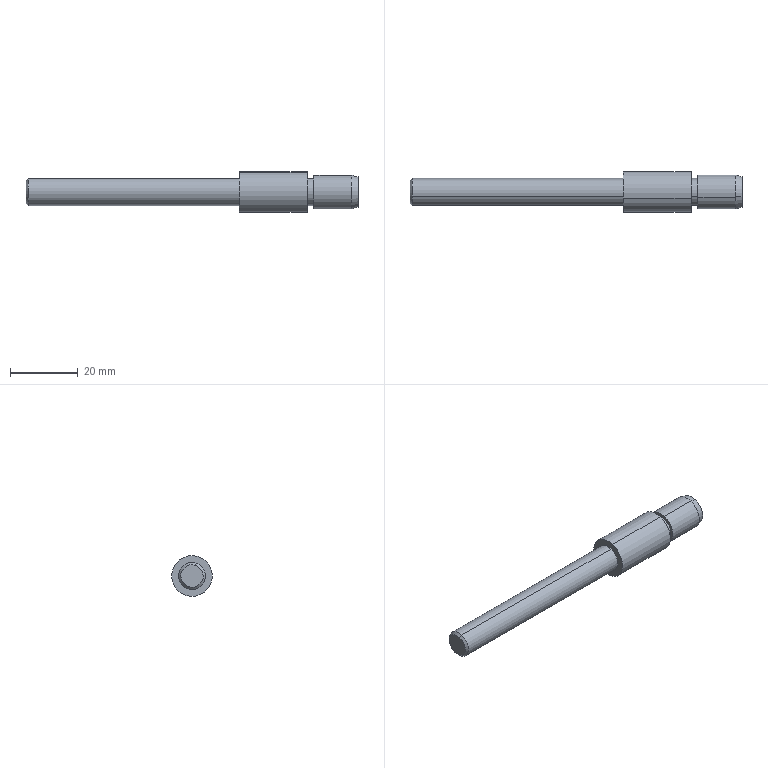Component | SolidWorks | 10Pin-1 | 1 solid | 17 faces | box 98 x 12 x 12 mm | volume 6529 mm3 | cylinder 8 | plane 5 | cone 4 | commonest cylinder face diameters 8 x4 10 x2 12 x2
STEP:
#1=COLOUR_RGB('',0.7922,0.8196,0.9333);
#2=FILL_AREA_STYLE_COLOUR('',#1);
#3=FILL_AREA_STYLE('',(#2));
#4=SURFACE_STYLE_FILL_AREA(#3);
#5=SURFACE_SIDE_STYLE('',(#4));
#6=SURFACE_STYLE_USAGE(.BOTH.,#5);
#7=PRESENTATION_STYLE_ASSIGNMENT((#6));
#8=CARTESIAN_POINT('',(-15.354,4.369,-0.1755));
#9=VERTEX_POINT('',#8);
#10=CARTESIAN_POINT('',(-15.354,4.291,0.07414));
#11=VERTEX_POINT('',#10);
#12=CARTESIAN_POINT('',(-15.354,4.33,-0.05068));
#13=DIRECTION('',(1.,0.,0.));
#14=DIRECTION('',(0.,0.3,-0.9539));
#15=AXIS2_PLACEMENT_3D('',#12,#13,#14);
#16=CIRCLE('',#15,0.1308);
#17=EDGE_CURVE('',#9,#11,#16,.T.);
#18=ORIENTED_EDGE('',*,*,#17,.T.);
#19=CARTESIAN_POINT('',(-15.328,4.283,0.09955));
#20=VERTEX_POINT('',#19);
#21=CARTESIAN_POINT('',(-15.354,4.291,0.07414));
#22=DIRECTION('',(0.7071,-0.2121,0.6745));
#23=VECTOR('',#22,39.37);
#24=LINE('',#21,#23);
#25=EDGE_CURVE('',#11,#20,#24,.T.);
#26=ORIENTED_EDGE('',*,*,#25,.T.);
#27=CARTESIAN_POINT('',(-15.328,4.377,-0.2009));
#28=VERTEX_POINT('',#27);
#29=CARTESIAN_POINT('',(-15.328,4.33,-0.05068));
#30=DIRECTION('',(1.,0.,0.));
#31=DIRECTION('',(0.,0.3,-0.9539));
#32=AXIS2_PLACEMENT_3D('',#29,#30,#31);
#33=CIRCLE('',#32,0.1575);
#34=EDGE_CURVE('',#28,#20,#33,.T.);
#35=ORIENTED_EDGE('',*,*,#34,.F.);
#36=CARTESIAN_POINT('',(-15.354,4.369,-0.1755));
#37=DIRECTION('',(0.7071,0.2121,-0.6745));
#38=VECTOR('',#37,39.37);
#39=LINE('',#36,#38);
#40=EDGE_CURVE('',#9,#28,#39,.T.);
#41=ORIENTED_EDGE('',*,*,#40,.F.);
#42=EDGE_LOOP('',(#18,#26,#35,#41));
#43=FACE_OUTER_BOUND('',#42,.T.);
#44=CARTESIAN_POINT('',(-15.354,4.33,-0.05068));
#45=DIRECTION('',(1.,0.,0.));
#46=DIRECTION('',(0.,0.3,-0.9539));
#47=AXIS2_PLACEMENT_3D('',#44,#45,#46);
#48=CONICAL_SURFACE('',#47,0.1308,0.7854);
#49=ADVANCED_FACE('',(#43),#48,.T.);
#50=CARTESIAN_POINT('',(-11.496,4.383,-0.2183));
#51=VERTEX_POINT('',#50);
#52=CARTESIAN_POINT('',(-11.496,4.277,0.117));
#53=VERTEX_POINT('',#52);
#54=CARTESIAN_POINT('',(-11.496,4.33,-0.05068));
#55=DIRECTION('',(1.,0.,0.));
#56=DIRECTION('',(0.,0.3,-0.9539));
#57=AXIS2_PLACEMENT_3D('',#54,#55,#56);
#58=CIRCLE('',#57,0.1758);
#59=EDGE_CURVE('',#51,#53,#58,.T.);
#60=ORIENTED_EDGE('',*,*,#59,.F.);
#61=CARTESIAN_POINT('',(-11.575,4.389,-0.2385));
#62=VERTEX_POINT('',#61);
#63=CARTESIAN_POINT('',(-11.496,4.383,-0.2183));
#64=DIRECTION('',(-0.9659,0.07764,-0.2469));
#65=VECTOR('',#64,39.37);
#66=LINE('',#63,#65);
#67=EDGE_CURVE('',#51,#62,#66,.T.);
#68=ORIENTED_EDGE('',*,*,#67,.T.);
#69=CARTESIAN_POINT('',(-11.575,4.271,0.1371));
#70=VERTEX_POINT('',#69);
#71=CARTESIAN_POINT('',(-11.575,4.33,-0.05068));
#72=DIRECTION('',(-1.,-0.,-0.));
#73=DIRECTION('',(0.,0.3,-0.9539));
#74=AXIS2_PLACEMENT_3D('',#71,#72,#73);
#75=CIRCLE('',#74,0.1969);
#76=EDGE_CURVE('',#70,#62,#75,.T.);
#77=ORIENTED_EDGE('',*,*,#76,.F.);
#78=CARTESIAN_POINT('',(-11.496,4.277,0.117));
#79=DIRECTION('',(-0.9659,-0.07764,0.2469));
#80=VECTOR('',#79,39.37);
#81=LINE('',#78,#80);
#82=EDGE_CURVE('',#53,#70,#81,.T.);
#83=ORIENTED_EDGE('',*,*,#82,.F.);
#84=EDGE_LOOP('',(#60,#68,#77,#83));
#85=FACE_OUTER_BOUND('',#84,.T.);
#86=CARTESIAN_POINT('',(-11.496,4.33,-0.05068));
#87=DIRECTION('',(-1.,-0.,-0.));
#88=DIRECTION('',(0.,-0.3,0.9539));
#89=AXIS2_PLACEMENT_3D('',#86,#87,#88);
#90=CONICAL_SURFACE('',#89,0.1758,0.2618);
#91=ADVANCED_FACE('',(#85),#90,.T.);
#92=ORIENTED_EDGE('',*,*,#76,.T.);
#93=CARTESIAN_POINT('',(-12.008,4.389,-0.2385));
#94=VERTEX_POINT('',#93);
#95=CARTESIAN_POINT('',(-11.496,4.389,-0.2385));
#96=DIRECTION('',(-1.,-0.,-0.));
#97=VECTOR('',#96,39.37);
#98=LINE('',#95,#97);
#99=EDGE_CURVE('',#62,#94,#98,.T.);
#100=ORIENTED_EDGE('',*,*,#99,.T.);
#101=CARTESIAN_POINT('',(-12.008,4.271,0.1371));
#102=VERTEX_POINT('',#101);
#103=CARTESIAN_POINT('',(-12.008,4.33,-0.05068));
#104=DIRECTION('',(1.,0.,0.));
#105=DIRECTION('',(0.,0.3,-0.9539));
#106=AXIS2_PLACEMENT_3D('',#103,#104,#105);
#107=CIRCLE('',#106,0.1969);
#108=EDGE_CURVE('',#94,#102,#107,.T.);
#109=ORIENTED_EDGE('',*,*,#108,.T.);
#110=CARTESIAN_POINT('',(-11.496,4.271,0.1371));
#111=DIRECTION('',(-1.,-0.,-0.));
#112=VECTOR('',#111,39.37);
#113=LINE('',#110,#112);
#114=EDGE_CURVE('',#70,#102,#113,.T.);
#115=ORIENTED_EDGE('',*,*,#114,.F.);
#116=EDGE_LOOP('',(#92,#100,#109,#115));
#117=FACE_OUTER_BOUND('',#116,.T.);
#118=CARTESIAN_POINT('',(-11.496,4.33,-0.05068));
#119=DIRECTION('',(-1.,-0.,-0.));
#120=DIRECTION('',(0.,-0.3,0.9539));
#121=AXIS2_PLACEMENT_3D('',#118,#119,#120);
#122=CYLINDRICAL_SURFACE('',#121,0.1969);
#123=ADVANCED_FACE('',(#117),#122,.T.);
#124=CARTESIAN_POINT('',(-12.008,4.377,-0.2009));
#125=VERTEX_POINT('',#124);
#126=CARTESIAN_POINT('',(-12.008,4.283,0.09955));
#127=VERTEX_POINT('',#126);
#128=CARTESIAN_POINT('',(-12.008,4.33,-0.05068));
#129=DIRECTION('',(1.,0.,0.));
#130=DIRECTION('',(0.,0.3,-0.9539));
#131=AXIS2_PLACEMENT_3D('',#128,#129,#130);
#132=CIRCLE('',#131,0.1575);
#133=EDGE_CURVE('',#125,#127,#132,.T.);
#134=ORIENTED_EDGE('',*,*,#133,.F.);
#135=CARTESIAN_POINT('',(-12.087,4.377,-0.2009));
#136=VERTEX_POINT('',#135);
#137=CARTESIAN_POINT('',(-12.008,4.377,-0.2009));
#138=DIRECTION('',(-1.,-0.,-0.));
#139=VECTOR('',#138,39.37);
#140=LINE('',#137,#139);
#141=EDGE_CURVE('',#125,#136,#140,.T.);
#142=ORIENTED_EDGE('',*,*,#141,.T.);
#143=CARTESIAN_POINT('',(-12.087,4.283,0.09955));
#144=VERTEX_POINT('',#143);
#145=CARTESIAN_POINT('',(-12.087,4.33,-0.05068));
#146=DIRECTION('',(1.,0.,0.));
#147=DIRECTION('',(0.,0.3,-0.9539));
#148=AXIS2_PLACEMENT_3D('',#145,#146,#147);
#149=CIRCLE('',#148,0.1575);
#150=EDGE_CURVE('',#136,#144,#149,.T.);
#151=ORIENTED_EDGE('',*,*,#150,.T.);
#152=CARTESIAN_POINT('',(-12.008,4.283,0.09955));
#153=DIRECTION('',(-1.,-0.,-0.));
#154=VECTOR('',#153,39.37);
#155=LINE('',#152,#154);
#156=EDGE_CURVE('',#127,#144,#155,.T.);
#157=ORIENTED_EDGE('',*,*,#156,.F.);
#158=EDGE_LOOP('',(#134,#142,#151,#157));
#159=FACE_OUTER_BOUND('',#158,.T.);
#160=CARTESIAN_POINT('',(-12.008,4.33,-0.05068));
#161=DIRECTION('',(-1.,-0.,-0.));
#162=DIRECTION('',(0.,-0.3,0.9539));
#163=AXIS2_PLACEMENT_3D('',#160,#161,#162);
#164=CYLINDRICAL_SURFACE('',#163,0.1575);
#165=ADVANCED_FACE('',(#159),#164,.T.);
#166=CARTESIAN_POINT('',(-12.087,4.401,-0.276));
#167=VERTEX_POINT('',#166);
#168=CARTESIAN_POINT('',(-12.087,4.259,0.1747));
#169=VERTEX_POINT('',#168);
#170=CARTESIAN_POINT('',(-12.087,4.33,-0.05068));
#171=DIRECTION('',(1.,0.,0.));
#172=DIRECTION('',(0.,0.3,-0.9539));
#173=AXIS2_PLACEMENT_3D('',#170,#171,#172);
#174=CIRCLE('',#173,0.2362);
#175=EDGE_CURVE('',#167,#169,#174,.T.);
#176=ORIENTED_EDGE('',*,*,#175,.F.);
#177=CARTESIAN_POINT('',(-12.874,4.401,-0.276));
#178=VERTEX_POINT('',#177);
#179=CARTESIAN_POINT('',(-12.087,4.401,-0.276));
#180=DIRECTION('',(-1.,-0.,-0.));
#181=VECTOR('',#180,39.37);
#182=LINE('',#179,#181);
#183=EDGE_CURVE('',#167,#178,#182,.T.);
#184=ORIENTED_EDGE('',*,*,#183,.T.);
#185=CARTESIAN_POINT('',(-12.874,4.259,0.1747));
#186=VERTEX_POINT('',#185);
#187=CARTESIAN_POINT('',(-12.874,4.33,-0.05068));
#188=DIRECTION('',(1.,0.,0.));
#189=DIRECTION('',(0.,0.3,-0.9539));
#190=AXIS2_PLACEMENT_3D('',#187,#188,#189);
#191=CIRCLE('',#190,0.2362);
#192=EDGE_CURVE('',#178,#186,#191,.T.);
#193=ORIENTED_EDGE('',*,*,#192,.T.);
#194=CARTESIAN_POINT('',(-12.087,4.259,0.1747));
#195=DIRECTION('',(-1.,-0.,-0.));
#196=VECTOR('',#195,39.37);
#197=LINE('',#194,#196);
#198=EDGE_CURVE('',#169,#186,#197,.T.);
#199=ORIENTED_EDGE('',*,*,#198,.F.);
#200=EDGE_LOOP('',(#176,#184,#193,#199));
#201=FACE_OUTER_BOUND('',#200,.T.);
#202=CARTESIAN_POINT('',(-12.087,4.33,-0.05068));
#203=DIRECTION('',(-1.,-0.,-0.));
#204=DIRECTION('',(0.,-0.3,0.9539));
#205=AXIS2_PLACEMENT_3D('',#202,#203,#204);
#206=CYLINDRICAL_SURFACE('',#205,0.2362);
#207=ADVANCED_FACE('',(#201),#206,.T.);
#208=CARTESIAN_POINT('',(-12.874,4.377,-0.2009));
#209=VERTEX_POINT('',#208);
#210=CARTESIAN_POINT('',(-12.874,4.283,0.09955));
#211=VERTEX_POINT('',#210);
#212=CARTESIAN_POINT('',(-12.874,4.33,-0.05068));
#213=DIRECTION('',(1.,0.,0.));
#214=DIRECTION('',(0.,0.3,-0.9539));
#215=AXIS2_PLACEMENT_3D('',#212,#213,#214);
#216=CIRCLE('',#215,0.1575);
#217=EDGE_CURVE('',#209,#211,#216,.T.);
#218=ORIENTED_EDGE('',*,*,#217,.F.);
#219=CARTESIAN_POINT('',(-12.874,4.377,-0.2009));
#220=DIRECTION('',(-1.,-0.,-0.));
#221=VECTOR('',#220,39.37);
#222=LINE('',#219,#221);
#223=EDGE_CURVE('',#209,#28,#222,.T.);
#224=ORIENTED_EDGE('',*,*,#223,.T.);
#225=ORIENTED_EDGE('',*,*,#34,.T.);
#226=CARTESIAN_POINT('',(-12.874,4.283,0.09955));
#227=DIRECTION('',(-1.,-0.,-0.));
#228=VECTOR('',#227,39.37);
#229=LINE('',#226,#228);
#230=EDGE_CURVE('',#211,#20,#229,.T.);
#231=ORIENTED_EDGE('',*,*,#230,.F.);
#232=EDGE_LOOP('',(#218,#224,#225,#231));
#233=FACE_OUTER_BOUND('',#232,.T.);
#234=CARTESIAN_POINT('',(-12.874,4.33,-0.05068));
#235=DIRECTION('',(-1.,-0.,-0.));
#236=DIRECTION('',(0.,-0.3,0.9539));
#237=AXIS2_PLACEMENT_3D('',#234,#235,#236);
#238=CYLINDRICAL_SURFACE('',#237,0.1575);
#239=ADVANCED_FACE('',(#233),#238,.T.);
#240=ORIENTED_EDGE('',*,*,#223,.F.);
#241=CARTESIAN_POINT('',(-12.874,4.33,-0.05068));
#242=DIRECTION('',(1.,0.,0.));
#243=DIRECTION('',(0.,0.3,-0.9539));
#244=AXIS2_PLACEMENT_3D('',#241,#242,#243);
#245=CIRCLE('',#244,0.1575);
#246=EDGE_CURVE('',#211,#209,#245,.T.);
#247=ORIENTED_EDGE('',*,*,#246,.F.);
#248=ORIENTED_EDGE('',*,*,#230,.T.);
#249=CARTESIAN_POINT('',(-15.328,4.33,-0.05068));
#250=DIRECTION('',(1.,0.,0.));
#251=DIRECTION('',(0.,0.3,-0.9539));
#252=AXIS2_PLACEMENT_3D('',#249,#250,#251);
#253=CIRCLE('',#252,0.1575);
#254=EDGE_CURVE('',#20,#28,#253,.T.);
#255=ORIENTED_EDGE('',*,*,#254,.T.);
#256=EDGE_LOOP('',(#240,#247,#248,#255));
#257=FACE_OUTER_BOUND('',#256,.T.);
#258=CARTESIAN_POINT('',(-12.874,4.33,-0.05068));
#259=DIRECTION('',(-1.,-0.,-0.));
#260=DIRECTION('',(0.,-0.3,0.9539));
#261=AXIS2_PLACEMENT_3D('',#258,#259,#260);
#262=CYLINDRICAL_SURFACE('',#261,0.1575);
#263=ADVANCED_FACE('',(#257),#262,.T.);
#264=ORIENTED_EDGE('',*,*,#183,.F.);
#265=CARTESIAN_POINT('',(-12.087,4.33,-0.05068));
#266=DIRECTION('',(1.,0.,0.));
#267=DIRECTION('',(0.,0.3,-0.9539));
#268=AXIS2_PLACEMENT_3D('',#265,#266,#267);
#269=CIRCLE('',#268,0.2362);
#270=EDGE_CURVE('',#169,#167,#269,.T.);
#271=ORIENTED_EDGE('',*,*,#270,.F.);
#272=ORIENTED_EDGE('',*,*,#198,.T.);
#273=CARTESIAN_POINT('',(-12.874,4.33,-0.05068));
#274=DIRECTION('',(1.,0.,0.));
#275=DIRECTION('',(0.,0.3,-0.9539));
#276=AXIS2_PLACEMENT_3D('',#273,#274,#275);
#277=CIRCLE('',#276,0.2362);
#278=EDGE_CURVE('',#186,#178,#277,.T.);
#279=ORIENTED_EDGE('',*,*,#278,.T.);
#280=EDGE_LOOP('',(#264,#271,#272,#279));
#281=FACE_OUTER_BOUND('',#280,.T.);
#282=CARTESIAN_POINT('',(-12.087,4.33,-0.05068));
#283=DIRECTION('',(-1.,-0.,-0.));
#284=DIRECTION('',(0.,-0.3,0.9539));
#285=AXIS2_PLACEMENT_3D('',#282,#283,#284);
#286=CYLINDRICAL_SURFACE('',#285,0.2362);
#287=ADVANCED_FACE('',(#281),#286,.T.);
#288=CARTESIAN_POINT('',(-12.087,4.33,-0.05068));
#289=DIRECTION('',(1.,0.,0.));
#290=DIRECTION('',(0.,0.3,-0.9539));
#291=AXIS2_PLACEMENT_3D('',#288,#289,#290);
#292=CIRCLE('',#291,0.1575);
#293=EDGE_CURVE('',#144,#136,#292,.T.);
#294=ORIENTED_EDGE('',*,*,#293,.F.);
#295=ORIENTED_EDGE('',*,*,#150,.F.);
#296=EDGE_LOOP('',(#294,#295));
#297=FACE_BOUND('',#296,.T.);
#298=ORIENTED_EDGE('',*,*,#270,.T.);
#299=ORIENTED_EDGE('',*,*,#175,.T.);
#300=EDGE_LOOP('',(#298,#299));
#301=FACE_OUTER_BOUND('',#300,.T.);
#302=CARTESIAN_POINT('',(-12.087,4.33,-0.05068));
#303=DIRECTION('',(1.,0.,0.));
#304=DIRECTION('',(0.,0.3,-0.9539));
#305=AXIS2_PLACEMENT_3D('',#302,#303,#304);
#306=PLANE('',#305);
#307=ADVANCED_FACE('',(#297,#301),#306,.T.);
#308=ORIENTED_EDGE('',*,*,#246,.T.);
#309=ORIENTED_EDGE('',*,*,#217,.T.);
#310=EDGE_LOOP('',(#308,#309));
#311=FACE_BOUND('',#310,.T.);
#312=ORIENTED_EDGE('',*,*,#278,.F.);
#313=ORIENTED_EDGE('',*,*,#192,.F.);
#314=EDGE_LOOP('',(#312,#313));
#315=FACE_OUTER_BOUND('',#314,.T.);
#316=CARTESIAN_POINT('',(-12.874,4.33,-0.05068));
#317=DIRECTION('',(1.,0.,0.));
#318=DIRECTION('',(0.,0.3,-0.9539));
#319=AXIS2_PLACEMENT_3D('',#316,#317,#318);
#320=PLANE('',#319);
#321=ADVANCED_FACE('',(#311,#315),#320,.F.);
#322=ORIENTED_EDGE('',*,*,#141,.F.);
#323=CARTESIAN_POINT('',(-12.008,4.33,-0.05068));
#324=DIRECTION('',(1.,0.,0.));
#325=DIRECTION('',(0.,0.3,-0.9539));
#326=AXIS2_PLACEMENT_3D('',#323,#324,#325);
#327=CIRCLE('',#326,0.1575);
#328=EDGE_CURVE('',#127,#125,#327,.T.);
#329=ORIENTED_EDGE('',*,*,#328,.F.);
#330=ORIENTED_EDGE('',*,*,#156,.T.);
#331=ORIENTED_EDGE('',*,*,#293,.T.);
#332=EDGE_LOOP('',(#322,#329,#330,#331));
#333=FACE_OUTER_BOUND('',#332,.T.);
#334=CARTESIAN_POINT('',(-12.008,4.33,-0.05068));
#335=DIRECTION('',(-1.,-0.,-0.));
#336=DIRECTION('',(0.,-0.3,0.9539));
#337=AXIS2_PLACEMENT_3D('',#334,#335,#336);
#338=CYLINDRICAL_SURFACE('',#337,0.1575);
#339=ADVANCED_FACE('',(#333),#338,.T.);
#340=ORIENTED_EDGE('',*,*,#99,.F.);
#341=CARTESIAN_POINT('',(-11.575,4.33,-0.05068));
#342=DIRECTION('',(-1.,-0.,-0.));
#343=DIRECTION('',(0.,0.3,-0.9539));
#344=AXIS2_PLACEMENT_3D('',#341,#342,#343);
#345=CIRCLE('',#344,0.1969);
#346=EDGE_CURVE('',#62,#70,#345,.T.);
#347=ORIENTED_EDGE('',*,*,#346,.T.);
#348=ORIENTED_EDGE('',*,*,#114,.T.);
#349=CARTESIAN_POINT('',(-12.008,4.33,-0.05068));
#350=DIRECTION('',(1.,0.,0.));
#351=DIRECTION('',(0.,0.3,-0.9539));
#352=AXIS2_PLACEMENT_3D('',#349,#350,#351);
#353=CIRCLE('',#352,0.1969);
#354=EDGE_CURVE('',#102,#94,#353,.T.);
#355=ORIENTED_EDGE('',*,*,#354,.T.);
#356=EDGE_LOOP('',(#340,#347,#348,#355));
#357=FACE_OUTER_BOUND('',#356,.T.);
#358=CARTESIAN_POINT('',(-11.496,4.33,-0.05068));
#359=DIRECTION('',(-1.,-0.,-0.));
#360=DIRECTION('',(0.,-0.3,0.9539));
#361=AXIS2_PLACEMENT_3D('',#358,#359,#360);
#362=CYLINDRICAL_SURFACE('',#361,0.1969);
#363=ADVANCED_FACE('',(#357),#362,.T.);
#364=CARTESIAN_POINT('',(-11.496,4.33,-0.05068));
#365=DIRECTION('',(1.,0.,0.));
#366=DIRECTION('',(0.,0.3,-0.9539));
#367=AXIS2_PLACEMENT_3D('',#364,#365,#366);
#368=CIRCLE('',#367,0.1758);
#369=EDGE_CURVE('',#53,#51,#368,.T.);
#370=ORIENTED_EDGE('',*,*,#369,.T.);
#371=ORIENTED_EDGE('',*,*,#59,.T.);
#372=EDGE_LOOP('',(#370,#371));
#373=FACE_OUTER_BOUND('',#372,.T.);
#374=CARTESIAN_POINT('',(-11.496,4.33,-0.05068));
#375=DIRECTION('',(1.,0.,0.));
#376=DIRECTION('',(0.,0.3,-0.9539));
#377=AXIS2_PLACEMENT_3D('',#374,#375,#376);
#378=PLANE('',#377);
#379=ADVANCED_FACE('',(#373),#378,.T.);
#380=ORIENTED_EDGE('',*,*,#328,.T.);
#381=ORIENTED_EDGE('',*,*,#133,.T.);
#382=EDGE_LOOP('',(#380,#381));
#383=FACE_BOUND('',#382,.T.);
#384=ORIENTED_EDGE('',*,*,#354,.F.);
#385=ORIENTED_EDGE('',*,*,#108,.F.);
#386=EDGE_LOOP('',(#384,#385));
#387=FACE_OUTER_BOUND('',#386,.T.);
#388=CARTESIAN_POINT('',(-12.008,4.33,-0.05068));
#389=DIRECTION('',(1.,0.,0.));
#390=DIRECTION('',(0.,0.3,-0.9539));
#391=AXIS2_PLACEMENT_3D('',#388,#389,#390);
#392=PLANE('',#391);
#393=ADVANCED_FACE('',(#383,#387),#392,.F.);
#394=ORIENTED_EDGE('',*,*,#67,.F.);
#395=ORIENTED_EDGE('',*,*,#369,.F.);
#396=ORIENTED_EDGE('',*,*,#82,.T.);
#397=ORIENTED_EDGE('',*,*,#346,.F.);
#398=EDGE_LOOP('',(#394,#395,#396,#397));
#399=FACE_OUTER_BOUND('',#398,.T.);
#400=CARTESIAN_POINT('',(-11.496,4.33,-0.05068));
#401=DIRECTION('',(-1.,-0.,-0.));
#402=DIRECTION('',(0.,-0.3,0.9539));
#403=AXIS2_PLACEMENT_3D('',#400,#401,#402);
#404=CONICAL_SURFACE('',#403,0.1758,0.2618);
#405=ADVANCED_FACE('',(#399),#404,.T.);
#406=ORIENTED_EDGE('',*,*,#25,.F.);
#407=CARTESIAN_POINT('',(-15.354,4.33,-0.05068));
#408=DIRECTION('',(1.,0.,0.));
#409=DIRECTION('',(0.,0.3,-0.9539));
#410=AXIS2_PLACEMENT_3D('',#407,#408,#409);
#411=CIRCLE('',#410,0.1308);
#412=EDGE_CURVE('',#11,#9,#411,.T.);
#413=ORIENTED_EDGE('',*,*,#412,.T.);
#414=ORIENTED_EDGE('',*,*,#40,.T.);
#415=ORIENTED_EDGE('',*,*,#254,.F.);
#416=EDGE_LOOP('',(#406,#413,#414,#415));
#417=FACE_OUTER_BOUND('',#416,.T.);
#418=CARTESIAN_POINT('',(-15.354,4.33,-0.05068));
#419=DIRECTION('',(1.,0.,0.));
#420=DIRECTION('',(0.,0.3,-0.9539));
#421=AXIS2_PLACEMENT_3D('',#418,#419,#420);
#422=CONICAL_SURFACE('',#421,0.1308,0.7854);
#423=ADVANCED_FACE('',(#417),#422,.T.);
#424=ORIENTED_EDGE('',*,*,#17,.F.);
#425=ORIENTED_EDGE('',*,*,#412,.F.);
#426=EDGE_LOOP('',(#424,#425));
#427=FACE_OUTER_BOUND('',#426,.T.);
#428=CARTESIAN_POINT('',(-15.354,4.33,-0.05068));
#429=DIRECTION('',(1.,0.,0.));
#430=DIRECTION('',(0.,0.3,-0.9539));
#431=AXIS2_PLACEMENT_3D('',#428,#429,#430);
#432=PLANE('',#431);
#433=ADVANCED_FACE('',(#427),#432,.F.);
#434=CLOSED_SHELL('',(#49,#91,#123,#165,#207,#239,#263,#287,#307,#321,#339,#363,#379,#393,#405,#423,#433));
#435=MANIFOLD_SOLID_BREP('',#434);
#436=STYLED_ITEM('',(#7),#435);
#437=PRESENTATION_LAYER_ASSIGNMENT('','',(#436));
#438=(LENGTH_UNIT()NAMED_UNIT(*)SI_UNIT($,.METRE.));
#439=LENGTH_MEASURE_WITH_UNIT(LENGTH_MEASURE(0.0254),#438);
#440=DIMENSIONAL_EXPONENTS(1.,0.,0.,0.,0.,0.,0.);
#441=(CONVERSION_BASED_UNIT('',#439)LENGTH_UNIT()NAMED_UNIT(#440));
#442=UNCERTAINTY_MEASURE_WITH_UNIT(LENGTH_MEASURE(0.00001),#441,'','');
#443=(NAMED_UNIT(*)PLANE_ANGLE_UNIT()SI_UNIT($,.RADIAN.));
#444=(NAMED_UNIT(*)SI_UNIT($,.STERADIAN.)SOLID_ANGLE_UNIT());
#445=(GEOMETRIC_REPRESENTATION_CONTEXT(3)GLOBAL_UNCERTAINTY_ASSIGNED_CONTEXT((#442))GLOBAL_UNIT_ASSIGNED_CONTEXT((#441,#443,#444))REPRESENTATION_CONTEXT('',''));
#446=MECHANICAL_DESIGN_GEOMETRIC_PRESENTATION_REPRESENTATION('',(#436),#445);
#447=CARTESIAN_POINT('',(0.,0.,0.));
#448=DIRECTION('',(0.,0.,1.));
#449=DIRECTION('',(1.,0.,0.));
#450=AXIS2_PLACEMENT_3D('',#447,#448,#449);
#451=(LENGTH_UNIT()NAMED_UNIT(*)SI_UNIT($,.METRE.));
#452=LENGTH_MEASURE_WITH_UNIT(LENGTH_MEASURE(0.0254),#451);
#453=DIMENSIONAL_EXPONENTS(1.,0.,0.,0.,0.,0.,0.);
#454=(CONVERSION_BASED_UNIT('',#452)LENGTH_UNIT()NAMED_UNIT(#453));
#455=UNCERTAINTY_MEASURE_WITH_UNIT(LENGTH_MEASURE(0.00001),#454,'','');
#456=(NAMED_UNIT(*)PLANE_ANGLE_UNIT()SI_UNIT($,.RADIAN.));
#457=(NAMED_UNIT(*)SI_UNIT($,.STERADIAN.)SOLID_ANGLE_UNIT());
#458=(GEOMETRIC_REPRESENTATION_CONTEXT(3)GLOBAL_UNCERTAINTY_ASSIGNED_CONTEXT((#455))GLOBAL_UNIT_ASSIGNED_CONTEXT((#454,#456,#457))REPRESENTATION_CONTEXT('',''));
#459=ADVANCED_BREP_SHAPE_REPRESENTATION('',(#435,#450),#458);